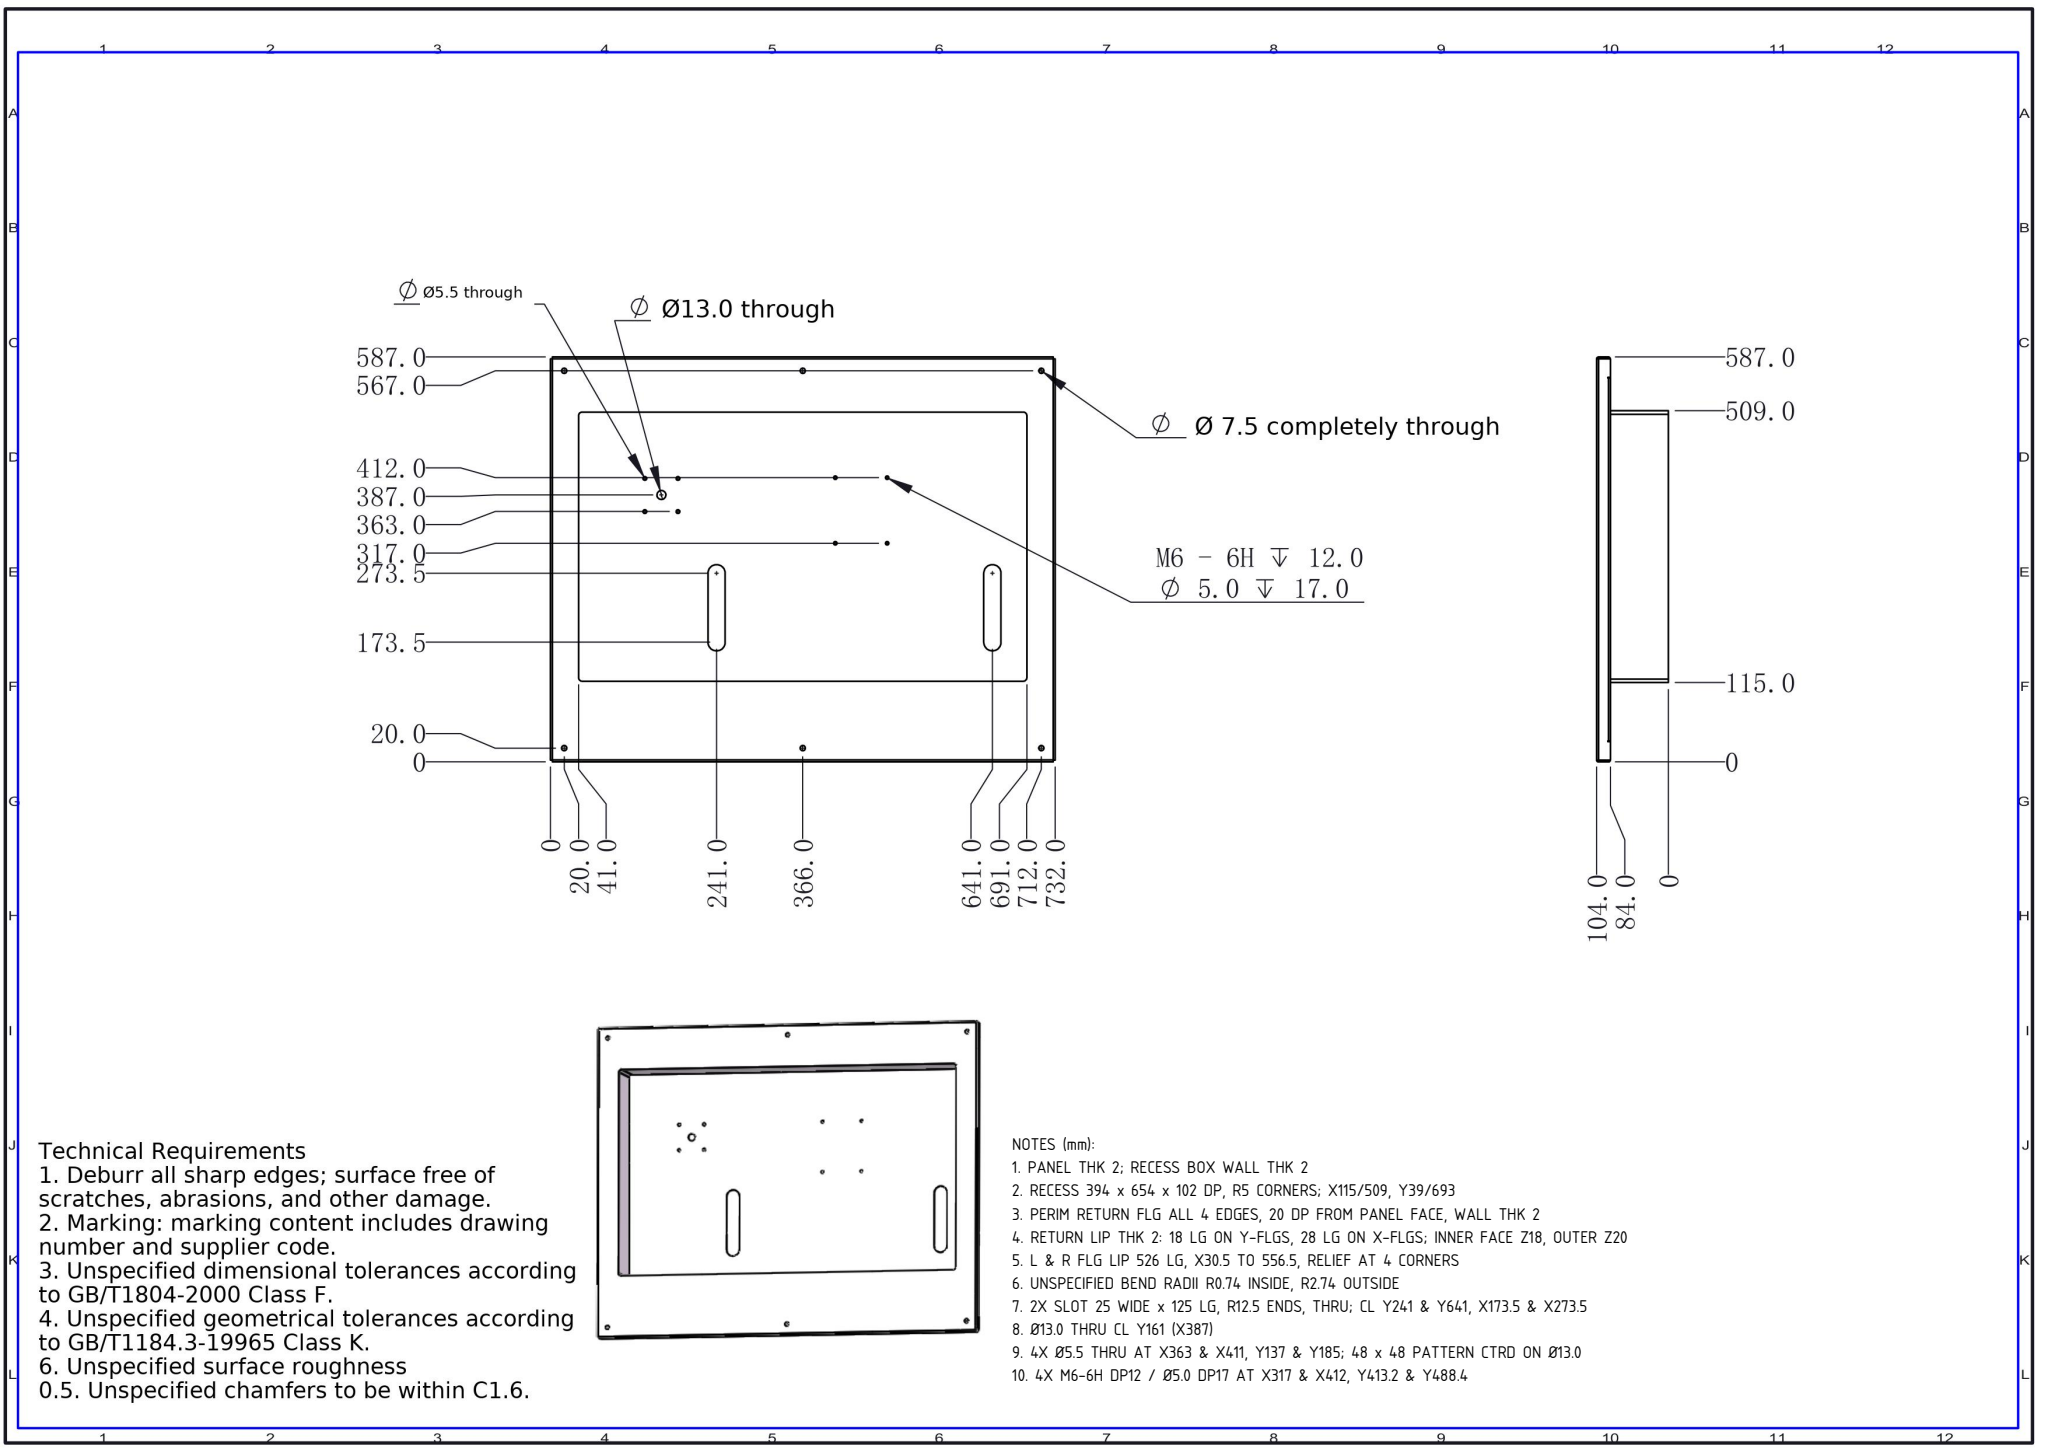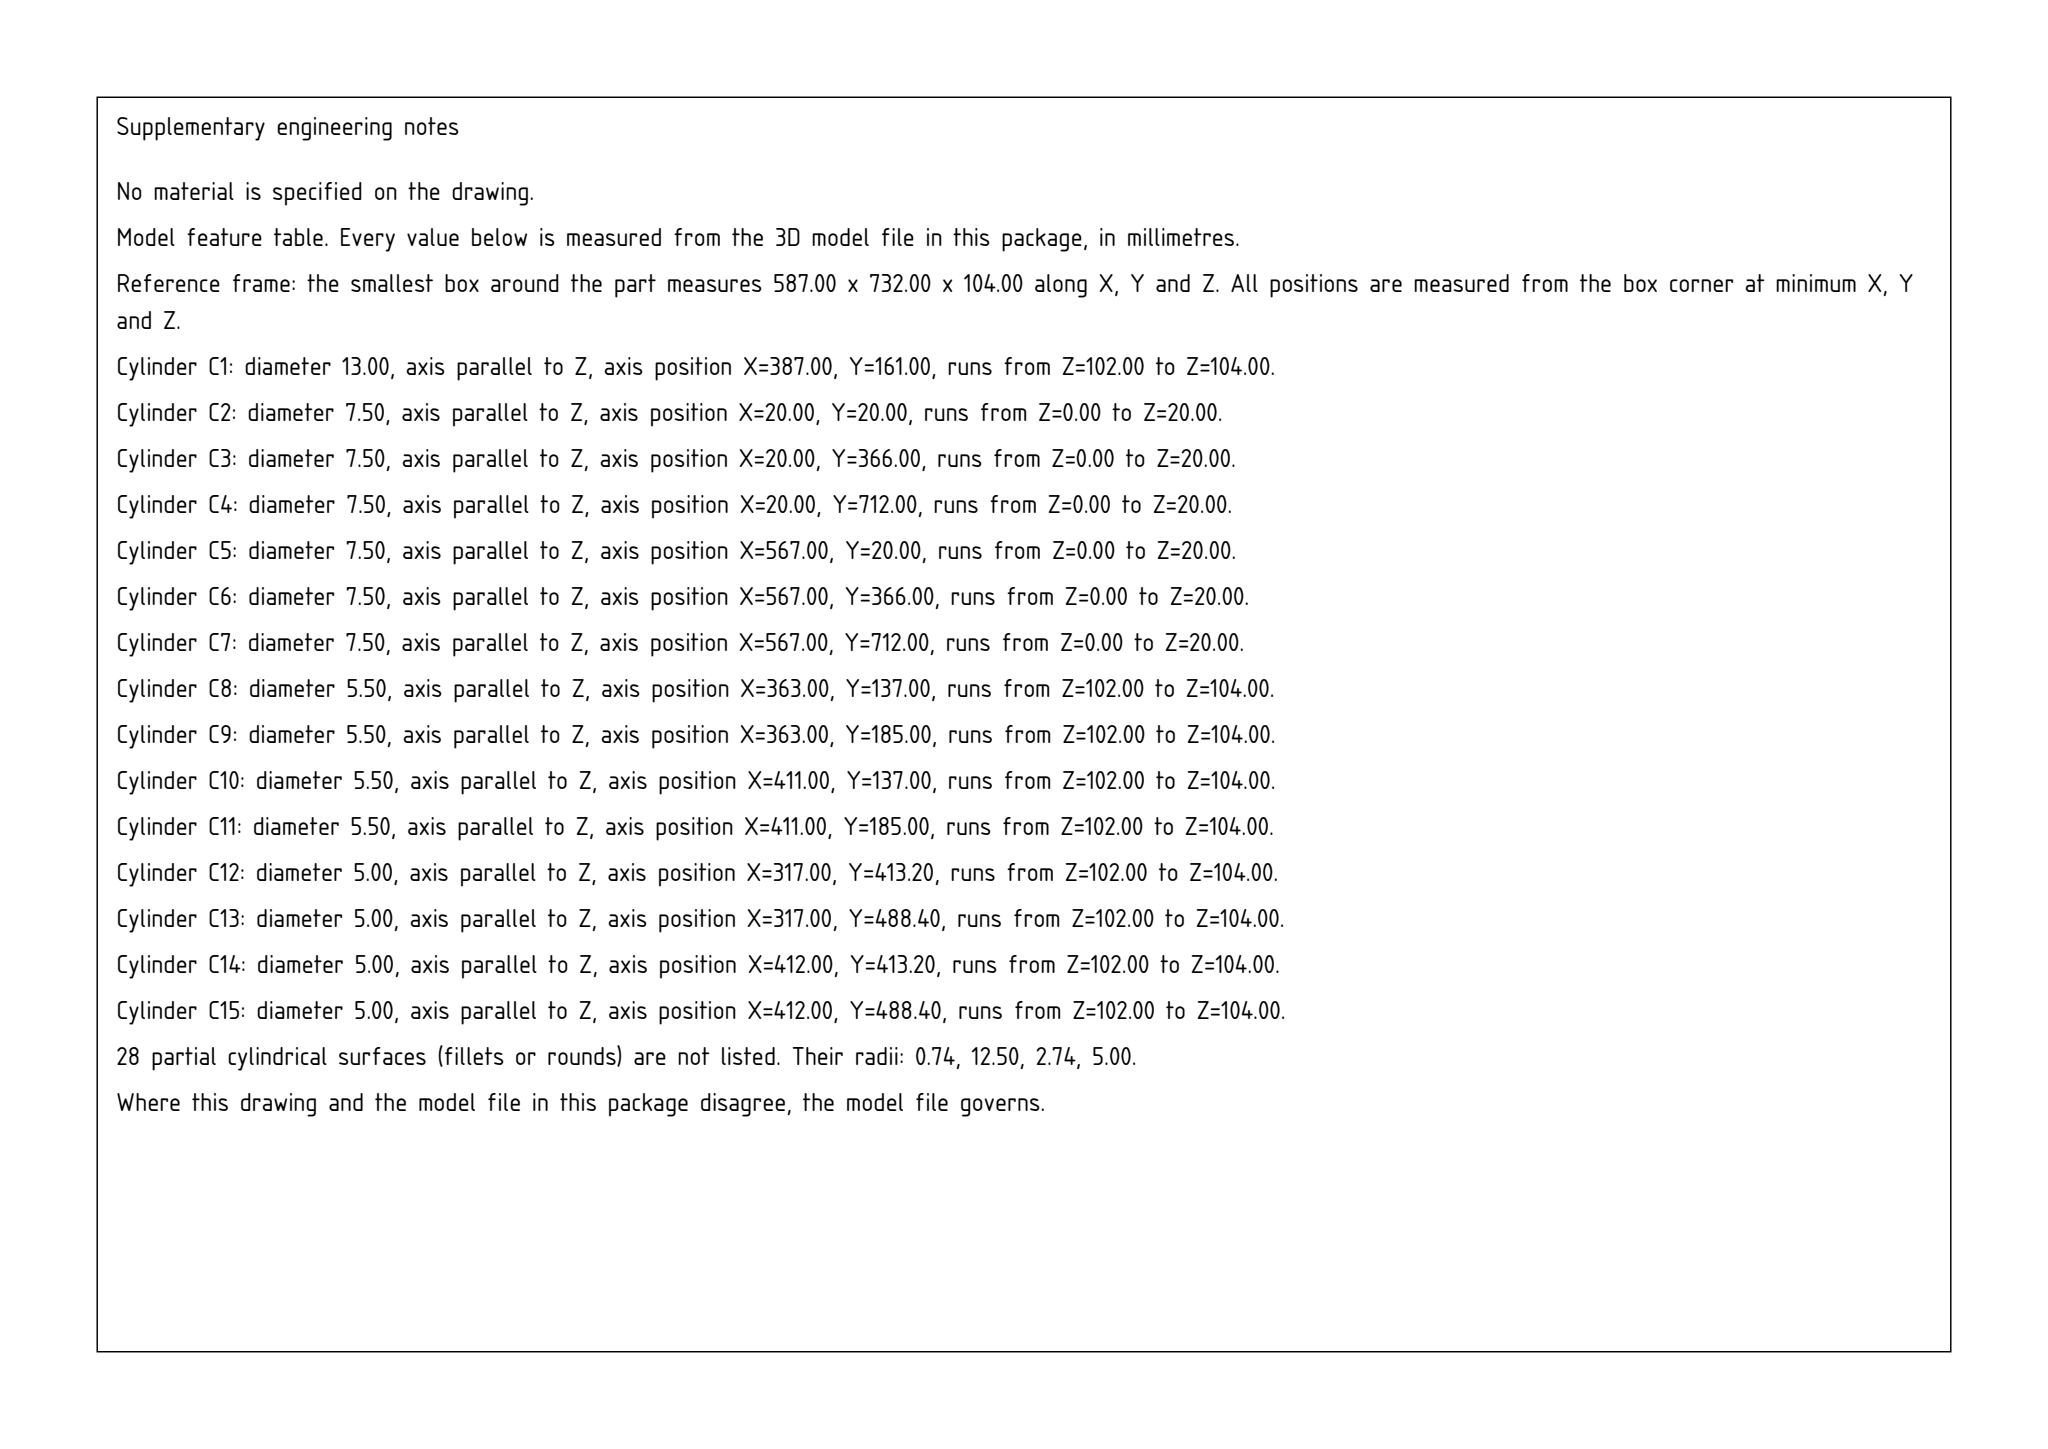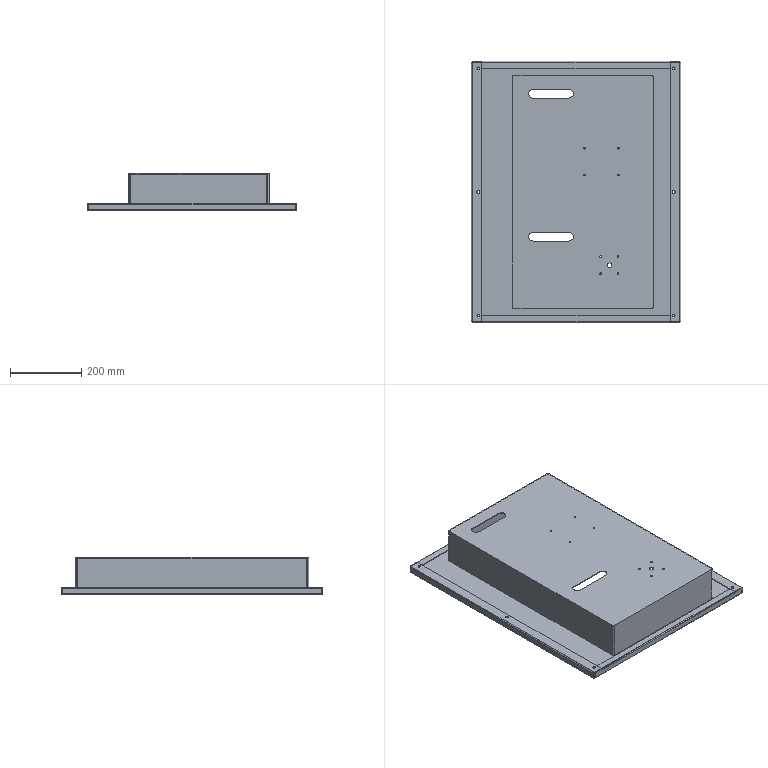Part | SolidWorks | mm | 1 solid | 156 faces | box 587 x 732 x 104 mm | volume 1477398 mm3 | plane 76 | cylinder 72 | spline 8 | commonest cylinder face diameters 7.5 x24 5 x8 5.5 x8 5.473 x8 1.473 x8 10 x8 25 x6 13 x2
Drawing notes:
PANEL THK 2; RECESS BOX WALL THK 2 | from the solid: z planes 0.02/2.02 & 102.02/104.02; inner box x117.02/507.02, y41.02/691.02 offset 2 from 115/509, 39/693
RECESS 394 x 654 x 102 DP, R5 CORNERS; X115/509, Y39/693 | from the solid: x planes 115.02 & 509.02, y planes 39.02 & 693.02, box z len 102; Ø10 corner cyls at (120,44),(504,688) = R5
PERIM RETURN FLG ALL 4 EDGES, 20 DP FROM PANEL FACE, WALL THK 2 | from the solid: z planes 0.02/2.02/18.02/20.02; x planes 2.02/585.02, y planes 2.02/730.02 (wall thk 2)
RETURN LIP THK 2: 18 LG ON Y-FLGS, 28 LG ON X-FLGS; INNER FACE Z18, OUTER Z20 | from the solid: lip free edges y=20.02 & 712.02 (18 from y2.02/730.02); x=30.02 & 557.02 (28 from x2.02/585.02); z=18.02/20.02
L & R FLG LIP 526 LG, X30.5 TO 556.5, RELIEF AT 4 CORNERS | from the solid: 2nd-bend cyl along x at (y=2.76,z=17.28) len 526.0; x planes 29.52/30.52/556.52/557.52; flange body x=2.73 to 584.31
UNSPECIFIED BEND RADII R0.74 INSIDE, R2.74 OUTSIDE | from the solid: flange edge cyls dia 1.473 (R0.7365) and dia 5.473 (R2.736)
2X SLOT 25 WIDE x 125 LG, R12.5 ENDS, THRU; CL Y241 & Y641, X173.5 & X273.5 | from the solid: Ø25 z-cyls at x=173.52 & 273.52, y=241.02 & 641.02, len 2.0 (ctr dist 100 + 25 width = 125 OAL)
Ø13.0 THRU CL Y161 (X387) | from the solid: cyl dia 13.0 axis z at [387.02, 161.02], length 2.0
4X Ø5.5 THRU AT X363 & X411, Y137 & Y185; 48 x 48 PATTERN CTRD ON Ø13.0 | from the solid: Ø5.5 z-cyls at x=363.02/411.02, y=137.02/185.02 (48 spacing); Ø13.0 at 387.02,161.02 = pattern center
4X M6-6H DP12 / Ø5.0 DP17 AT X317 & X412, Y413.2 & Y488.4 | from the solid: Ø5.0 z-cyls at x=317.02 & 412.02, y=413.22 & 488.42